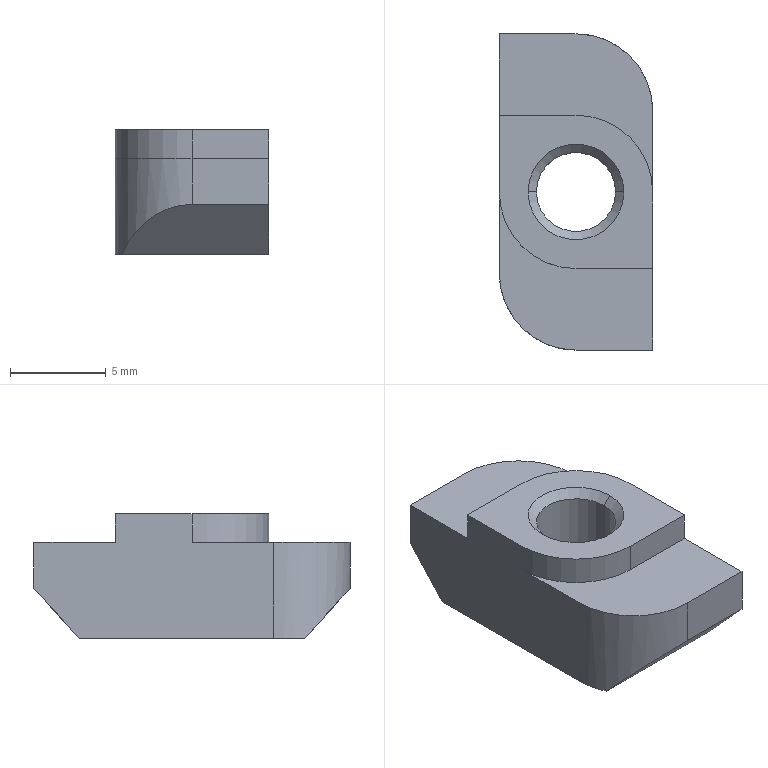Component | SolidWorks | 170423A4-AHC21-308-M5-1 | 1 solid | 22 faces | box 8 x 16.5 x 6.5 mm | volume 584 mm3 | plane 12 | cylinder 6 | cone 4 | commonest cylinder face diameters 8 x4 4.134 x2
STEP:
#1=COLOUR_RGB('',0.7922,0.8196,0.9333);
#2=FILL_AREA_STYLE_COLOUR('',#1);
#3=FILL_AREA_STYLE('',(#2));
#4=SURFACE_STYLE_FILL_AREA(#3);
#5=SURFACE_SIDE_STYLE('',(#4));
#6=SURFACE_STYLE_USAGE(.BOTH.,#5);
#7=PRESENTATION_STYLE_ASSIGNMENT((#6));
#8=CARTESIAN_POINT('',(-7.605,-0.8381,17.989));
#9=VERTEX_POINT('',#8);
#10=CARTESIAN_POINT('',(-7.768,-0.8381,17.989));
#11=VERTEX_POINT('',#10);
#12=CARTESIAN_POINT('',(-7.687,-0.8381,17.989));
#13=DIRECTION('',(0.,0.,-1.));
#14=DIRECTION('',(-1.,0.,0.));
#15=AXIS2_PLACEMENT_3D('',#12,#13,#14);
#16=CIRCLE('',#15,0.08138);
#17=EDGE_CURVE('',#9,#11,#16,.T.);
#18=ORIENTED_EDGE('',*,*,#17,.F.);
#19=CARTESIAN_POINT('',(-7.588,-0.8381,17.972));
#20=VERTEX_POINT('',#19);
#21=CARTESIAN_POINT('',(-7.588,-0.8381,17.972));
#22=DIRECTION('',(0.7071,0.,-0.7071));
#23=VECTOR('',#22,39.37);
#24=LINE('',#21,#23);
#25=EDGE_CURVE('',#9,#20,#24,.T.);
#26=ORIENTED_EDGE('',*,*,#25,.T.);
#27=CARTESIAN_POINT('',(-7.785,-0.8381,17.972));
#28=VERTEX_POINT('',#27);
#29=CARTESIAN_POINT('',(-7.687,-0.8381,17.972));
#30=DIRECTION('',(0.,0.,-1.));
#31=DIRECTION('',(-1.,0.,0.));
#32=AXIS2_PLACEMENT_3D('',#29,#30,#31);
#33=CIRCLE('',#32,0.09843);
#34=EDGE_CURVE('',#20,#28,#33,.T.);
#35=ORIENTED_EDGE('',*,*,#34,.T.);
#36=CARTESIAN_POINT('',(-7.785,-0.8381,17.972));
#37=DIRECTION('',(-0.7071,-0.,-0.7071));
#38=VECTOR('',#37,39.37);
#39=LINE('',#36,#38);
#40=EDGE_CURVE('',#11,#28,#39,.T.);
#41=ORIENTED_EDGE('',*,*,#40,.F.);
#42=EDGE_LOOP('',(#18,#26,#35,#41));
#43=FACE_OUTER_BOUND('',#42,.T.);
#44=CARTESIAN_POINT('',(-7.687,-0.8381,17.972));
#45=DIRECTION('',(0.,0.,-1.));
#46=DIRECTION('',(-1.,0.,0.));
#47=AXIS2_PLACEMENT_3D('',#44,#45,#46);
#48=CONICAL_SURFACE('',#47,0.09843,0.7854);
#49=ADVANCED_FACE('',(#43),#48,.F.);
#50=ORIENTED_EDGE('',*,*,#17,.T.);
#51=CARTESIAN_POINT('',(-7.768,-0.8381,18.211));
#52=VERTEX_POINT('',#51);
#53=CARTESIAN_POINT('',(-7.768,-0.8381,17.972));
#54=DIRECTION('',(-0.,-0.,1.));
#55=VECTOR('',#54,39.37);
#56=LINE('',#53,#55);
#57=EDGE_CURVE('',#11,#52,#56,.T.);
#58=ORIENTED_EDGE('',*,*,#57,.T.);
#59=CARTESIAN_POINT('',(-7.605,-0.8381,18.211));
#60=VERTEX_POINT('',#59);
#61=CARTESIAN_POINT('',(-7.687,-0.8381,18.211));
#62=DIRECTION('',(0.,0.,-1.));
#63=DIRECTION('',(1.,0.,0.));
#64=AXIS2_PLACEMENT_3D('',#61,#62,#63);
#65=CIRCLE('',#64,0.08138);
#66=EDGE_CURVE('',#60,#52,#65,.T.);
#67=ORIENTED_EDGE('',*,*,#66,.F.);
#68=CARTESIAN_POINT('',(-7.605,-0.8381,17.972));
#69=DIRECTION('',(-0.,-0.,1.));
#70=VECTOR('',#69,39.37);
#71=LINE('',#68,#70);
#72=EDGE_CURVE('',#9,#60,#71,.T.);
#73=ORIENTED_EDGE('',*,*,#72,.F.);
#74=EDGE_LOOP('',(#50,#58,#67,#73));
#75=FACE_OUTER_BOUND('',#74,.T.);
#76=CARTESIAN_POINT('',(-7.687,-0.8381,17.972));
#77=DIRECTION('',(-0.,-0.,1.));
#78=DIRECTION('',(1.,0.,0.));
#79=AXIS2_PLACEMENT_3D('',#76,#77,#78);
#80=CYLINDRICAL_SURFACE('',#79,0.08138);
#81=ADVANCED_FACE('',(#75),#80,.F.);
#82=ORIENTED_EDGE('',*,*,#66,.T.);
#83=CARTESIAN_POINT('',(-7.785,-0.8381,18.228));
#84=VERTEX_POINT('',#83);
#85=CARTESIAN_POINT('',(-7.785,-0.8381,18.228));
#86=DIRECTION('',(-0.7071,0.,0.7071));
#87=VECTOR('',#86,39.37);
#88=LINE('',#85,#87);
#89=EDGE_CURVE('',#52,#84,#88,.T.);
#90=ORIENTED_EDGE('',*,*,#89,.T.);
#91=CARTESIAN_POINT('',(-7.588,-0.8381,18.228));
#92=VERTEX_POINT('',#91);
#93=CARTESIAN_POINT('',(-7.687,-0.8381,18.228));
#94=DIRECTION('',(0.,0.,-1.));
#95=DIRECTION('',(1.,0.,0.));
#96=AXIS2_PLACEMENT_3D('',#93,#94,#95);
#97=CIRCLE('',#96,0.09843);
#98=EDGE_CURVE('',#92,#84,#97,.T.);
#99=ORIENTED_EDGE('',*,*,#98,.F.);
#100=CARTESIAN_POINT('',(-7.588,-0.8381,18.228));
#101=DIRECTION('',(0.7071,0.,0.7071));
#102=VECTOR('',#101,39.37);
#103=LINE('',#100,#102);
#104=EDGE_CURVE('',#60,#92,#103,.T.);
#105=ORIENTED_EDGE('',*,*,#104,.F.);
#106=EDGE_LOOP('',(#82,#90,#99,#105));
#107=FACE_OUTER_BOUND('',#106,.T.);
#108=CARTESIAN_POINT('',(-7.687,-0.8381,18.228));
#109=DIRECTION('',(-0.,-0.,1.));
#110=DIRECTION('',(1.,0.,0.));
#111=AXIS2_PLACEMENT_3D('',#108,#109,#110);
#112=CONICAL_SURFACE('',#111,0.09843,0.7854);
#113=ADVANCED_FACE('',(#107),#112,.F.);
#114=CARTESIAN_POINT('',(-7.529,-1.07,17.972));
#115=VERTEX_POINT('',#114);
#116=CARTESIAN_POINT('',(-7.529,-1.163,18.075));
#117=VERTEX_POINT('',#116);
#118=CARTESIAN_POINT('',(-7.529,-1.034,17.933));
#119=DIRECTION('',(0.,-0.6734,0.7393));
#120=VECTOR('',#119,39.37);
#121=LINE('',#118,#120);
#122=EDGE_CURVE('',#115,#117,#121,.T.);
#123=ORIENTED_EDGE('',*,*,#122,.F.);
#124=CARTESIAN_POINT('',(-7.529,-0.6708,17.972));
#125=VERTEX_POINT('',#124);
#126=CARTESIAN_POINT('',(-7.529,-0.6708,17.972));
#127=DIRECTION('',(-0.,1.,0.));
#128=VECTOR('',#127,39.37);
#129=LINE('',#126,#128);
#130=EDGE_CURVE('',#115,#125,#129,.T.);
#131=ORIENTED_EDGE('',*,*,#130,.T.);
#132=CARTESIAN_POINT('',(-7.529,-0.6708,18.169));
#133=VERTEX_POINT('',#132);
#134=CARTESIAN_POINT('',(-7.529,-0.6708,18.169));
#135=DIRECTION('',(0.,0.,-1.));
#136=VECTOR('',#135,39.37);
#137=LINE('',#134,#136);
#138=EDGE_CURVE('',#133,#125,#137,.T.);
#139=ORIENTED_EDGE('',*,*,#138,.F.);
#140=CARTESIAN_POINT('',(-7.529,-0.8381,18.169));
#141=VERTEX_POINT('',#140);
#142=CARTESIAN_POINT('',(-7.529,-1.163,18.169));
#143=DIRECTION('',(-0.,1.,0.));
#144=VECTOR('',#143,39.37);
#145=LINE('',#142,#144);
#146=EDGE_CURVE('',#141,#133,#145,.T.);
#147=ORIENTED_EDGE('',*,*,#146,.F.);
#148=CARTESIAN_POINT('',(-7.529,-0.8381,18.228));
#149=VERTEX_POINT('',#148);
#150=CARTESIAN_POINT('',(-7.529,-0.8381,18.228));
#151=DIRECTION('',(0.,0.,-1.));
#152=VECTOR('',#151,39.37);
#153=LINE('',#150,#152);
#154=EDGE_CURVE('',#149,#141,#153,.T.);
#155=ORIENTED_EDGE('',*,*,#154,.F.);
#156=CARTESIAN_POINT('',(-7.529,-0.9956,18.228));
#157=VERTEX_POINT('',#156);
#158=CARTESIAN_POINT('',(-7.529,-1.163,18.228));
#159=DIRECTION('',(-0.,1.,0.));
#160=VECTOR('',#159,39.37);
#161=LINE('',#158,#160);
#162=EDGE_CURVE('',#157,#149,#161,.T.);
#163=ORIENTED_EDGE('',*,*,#162,.F.);
#164=CARTESIAN_POINT('',(-7.529,-0.9956,18.169));
#165=VERTEX_POINT('',#164);
#166=CARTESIAN_POINT('',(-7.529,-0.9956,18.228));
#167=DIRECTION('',(0.,0.,-1.));
#168=VECTOR('',#167,39.37);
#169=LINE('',#166,#168);
#170=EDGE_CURVE('',#157,#165,#169,.T.);
#171=ORIENTED_EDGE('',*,*,#170,.T.);
#172=CARTESIAN_POINT('',(-7.529,-1.163,18.169));
#173=VERTEX_POINT('',#172);
#174=CARTESIAN_POINT('',(-7.529,-1.163,18.169));
#175=DIRECTION('',(-0.,1.,0.));
#176=VECTOR('',#175,39.37);
#177=LINE('',#174,#176);
#178=EDGE_CURVE('',#173,#165,#177,.T.);
#179=ORIENTED_EDGE('',*,*,#178,.F.);
#180=CARTESIAN_POINT('',(-7.529,-1.163,18.169));
#181=DIRECTION('',(-0.,-0.,1.));
#182=VECTOR('',#181,39.37);
#183=LINE('',#180,#182);
#184=EDGE_CURVE('',#117,#173,#183,.T.);
#185=ORIENTED_EDGE('',*,*,#184,.F.);
#186=EDGE_LOOP('',(#123,#131,#139,#147,#155,#163,#171,#179,#185));
#187=FACE_OUTER_BOUND('',#186,.T.);
#188=CARTESIAN_POINT('',(-7.529,-1.163,18.169));
#189=DIRECTION('',(-1.,-0.,-0.));
#190=DIRECTION('',(0.,-1.,-0.));
#191=AXIS2_PLACEMENT_3D('',#188,#189,#190);
#192=PLANE('',#191);
#193=ADVANCED_FACE('',(#187),#192,.F.);
#194=CARTESIAN_POINT('',(-7.687,-0.8381,17.972));
#195=DIRECTION('',(0.,0.,-1.));
#196=DIRECTION('',(-1.,0.,0.));
#197=AXIS2_PLACEMENT_3D('',#194,#195,#196);
#198=CIRCLE('',#197,0.09843);
#199=EDGE_CURVE('',#28,#20,#198,.T.);
#200=ORIENTED_EDGE('',*,*,#199,.F.);
#201=ORIENTED_EDGE('',*,*,#34,.F.);
#202=EDGE_LOOP('',(#200,#201));
#203=FACE_BOUND('',#202,.T.);
#204=CARTESIAN_POINT('',(-7.844,-0.6066,17.972));
#205=VERTEX_POINT('',#204);
#206=CARTESIAN_POINT('',(-7.844,-1.005,17.972));
#207=VERTEX_POINT('',#206);
#208=CARTESIAN_POINT('',(-7.844,-0.6708,17.972));
#209=DIRECTION('',(0.,-1.,-0.));
#210=VECTOR('',#209,39.37);
#211=LINE('',#208,#210);
#212=EDGE_CURVE('',#205,#207,#211,.T.);
#213=ORIENTED_EDGE('',*,*,#212,.F.);
#214=CARTESIAN_POINT('',(-7.543,-0.6066,17.972));
#215=VERTEX_POINT('',#214);
#216=CARTESIAN_POINT('',(-7.687,-0.6066,17.972));
#217=DIRECTION('',(1.,0.,0.));
#218=VECTOR('',#217,39.37);
#219=LINE('',#216,#218);
#220=EDGE_CURVE('',#205,#215,#219,.T.);
#221=ORIENTED_EDGE('',*,*,#220,.T.);
#222=CARTESIAN_POINT('',(-7.687,-0.6708,17.972));
#223=DIRECTION('',(-0.,-0.,1.));
#224=DIRECTION('',(1.,0.,0.));
#225=AXIS2_PLACEMENT_3D('',#222,#223,#224);
#226=CIRCLE('',#225,0.1575);
#227=EDGE_CURVE('',#125,#215,#226,.T.);
#228=ORIENTED_EDGE('',*,*,#227,.F.);
#229=ORIENTED_EDGE('',*,*,#130,.F.);
#230=CARTESIAN_POINT('',(-7.831,-1.07,17.972));
#231=VERTEX_POINT('',#230);
#232=CARTESIAN_POINT('',(-7.687,-1.07,17.972));
#233=DIRECTION('',(-1.,-0.,-0.));
#234=VECTOR('',#233,39.37);
#235=LINE('',#232,#234);
#236=EDGE_CURVE('',#115,#231,#235,.T.);
#237=ORIENTED_EDGE('',*,*,#236,.T.);
#238=CARTESIAN_POINT('',(-7.687,-1.005,17.972));
#239=DIRECTION('',(-0.,-0.,1.));
#240=DIRECTION('',(1.,0.,0.));
#241=AXIS2_PLACEMENT_3D('',#238,#239,#240);
#242=CIRCLE('',#241,0.1575);
#243=EDGE_CURVE('',#207,#231,#242,.T.);
#244=ORIENTED_EDGE('',*,*,#243,.F.);
#245=EDGE_LOOP('',(#213,#221,#228,#229,#237,#244));
#246=FACE_OUTER_BOUND('',#245,.T.);
#247=CARTESIAN_POINT('',(-7.687,-0.6708,17.972));
#248=DIRECTION('',(-0.,-0.,1.));
#249=DIRECTION('',(1.,0.,0.));
#250=AXIS2_PLACEMENT_3D('',#247,#248,#249);
#251=PLANE('',#250);
#252=ADVANCED_FACE('',(#203,#246),#251,.F.);
#253=ORIENTED_EDGE('',*,*,#25,.F.);
#254=CARTESIAN_POINT('',(-7.687,-0.8381,17.989));
#255=DIRECTION('',(0.,0.,-1.));
#256=DIRECTION('',(-1.,0.,0.));
#257=AXIS2_PLACEMENT_3D('',#254,#255,#256);
#258=CIRCLE('',#257,0.08138);
#259=EDGE_CURVE('',#11,#9,#258,.T.);
#260=ORIENTED_EDGE('',*,*,#259,.F.);
#261=ORIENTED_EDGE('',*,*,#40,.T.);
#262=ORIENTED_EDGE('',*,*,#199,.T.);
#263=EDGE_LOOP('',(#253,#260,#261,#262));
#264=FACE_OUTER_BOUND('',#263,.T.);
#265=CARTESIAN_POINT('',(-7.687,-0.8381,17.972));
#266=DIRECTION('',(0.,0.,-1.));
#267=DIRECTION('',(-1.,0.,0.));
#268=AXIS2_PLACEMENT_3D('',#265,#266,#267);
#269=CONICAL_SURFACE('',#268,0.09843,0.7854);
#270=ADVANCED_FACE('',(#264),#269,.F.);
#271=CARTESIAN_POINT('',(-7.844,-0.5133,18.075));
#272=VERTEX_POINT('',#271);
#273=CARTESIAN_POINT('',(-7.844,-0.5133,18.169));
#274=VERTEX_POINT('',#273);
#275=CARTESIAN_POINT('',(-7.844,-0.5133,18.169));
#276=DIRECTION('',(-0.,-0.,1.));
#277=VECTOR('',#276,39.37);
#278=LINE('',#275,#277);
#279=EDGE_CURVE('',#272,#274,#278,.T.);
#280=ORIENTED_EDGE('',*,*,#279,.F.);
#281=CARTESIAN_POINT('',(-7.844,-0.4775,18.114));
#282=DIRECTION('',(0.,-0.6734,-0.7393));
#283=VECTOR('',#282,39.37);
#284=LINE('',#281,#283);
#285=EDGE_CURVE('',#272,#205,#284,.T.);
#286=ORIENTED_EDGE('',*,*,#285,.T.);
#287=ORIENTED_EDGE('',*,*,#212,.T.);
#288=CARTESIAN_POINT('',(-7.844,-1.005,18.169));
#289=VERTEX_POINT('',#288);
#290=CARTESIAN_POINT('',(-7.844,-1.005,18.169));
#291=DIRECTION('',(0.,0.,-1.));
#292=VECTOR('',#291,39.37);
#293=LINE('',#290,#292);
#294=EDGE_CURVE('',#289,#207,#293,.T.);
#295=ORIENTED_EDGE('',*,*,#294,.F.);
#296=CARTESIAN_POINT('',(-7.844,-0.8381,18.169));
#297=VERTEX_POINT('',#296);
#298=CARTESIAN_POINT('',(-7.844,-0.5133,18.169));
#299=DIRECTION('',(-0.,-1.,-0.));
#300=VECTOR('',#299,39.37);
#301=LINE('',#298,#300);
#302=EDGE_CURVE('',#297,#289,#301,.T.);
#303=ORIENTED_EDGE('',*,*,#302,.F.);
#304=CARTESIAN_POINT('',(-7.844,-0.8381,18.228));
#305=VERTEX_POINT('',#304);
#306=CARTESIAN_POINT('',(-7.844,-0.8381,18.228));
#307=DIRECTION('',(0.,0.,-1.));
#308=VECTOR('',#307,39.37);
#309=LINE('',#306,#308);
#310=EDGE_CURVE('',#305,#297,#309,.T.);
#311=ORIENTED_EDGE('',*,*,#310,.F.);
#312=CARTESIAN_POINT('',(-7.844,-0.6806,18.228));
#313=VERTEX_POINT('',#312);
#314=CARTESIAN_POINT('',(-7.844,-0.5133,18.228));
#315=DIRECTION('',(-0.,-1.,-0.));
#316=VECTOR('',#315,39.37);
#317=LINE('',#314,#316);
#318=EDGE_CURVE('',#313,#305,#317,.T.);
#319=ORIENTED_EDGE('',*,*,#318,.F.);
#320=CARTESIAN_POINT('',(-7.844,-0.6806,18.169));
#321=VERTEX_POINT('',#320);
#322=CARTESIAN_POINT('',(-7.844,-0.6806,18.228));
#323=DIRECTION('',(0.,0.,-1.));
#324=VECTOR('',#323,39.37);
#325=LINE('',#322,#324);
#326=EDGE_CURVE('',#313,#321,#325,.T.);
#327=ORIENTED_EDGE('',*,*,#326,.T.);
#328=CARTESIAN_POINT('',(-7.844,-0.5133,18.169));
#329=DIRECTION('',(-0.,-1.,-0.));
#330=VECTOR('',#329,39.37);
#331=LINE('',#328,#330);
#332=EDGE_CURVE('',#274,#321,#331,.T.);
#333=ORIENTED_EDGE('',*,*,#332,.F.);
#334=EDGE_LOOP('',(#280,#286,#287,#295,#303,#311,#319,#327,#333));
#335=FACE_OUTER_BOUND('',#334,.T.);
#336=CARTESIAN_POINT('',(-7.844,-0.5133,18.169));
#337=DIRECTION('',(1.,-0.,0.));
#338=DIRECTION('',(0.,1.,0.));
#339=AXIS2_PLACEMENT_3D('',#336,#337,#338);
#340=PLANE('',#339);
#341=ADVANCED_FACE('',(#335),#340,.F.);
#342=CARTESIAN_POINT('',(-7.687,-0.5133,18.075));
#343=VERTEX_POINT('',#342);
#344=CARTESIAN_POINT('',(-7.687,-0.5133,18.075));
#345=CARTESIAN_POINT('',(-7.623,-0.5133,18.075));
#346=CARTESIAN_POINT('',(-7.569,-0.5481,18.037));
#347=CARTESIAN_POINT('',(-7.543,-0.6066,17.972));
#348=(BOUNDED_CURVE()B_SPLINE_CURVE(3,(#344,#345,#346,#347),.UNSPECIFIED.,.F.,.T.)B_SPLINE_CURVE_WITH_KNOTS((4,4),(0.,1.151),.UNSPECIFIED.)CURVE()GEOMETRIC_REPRESENTATION_ITEM()RATIONAL_B_SPLINE_CURVE((1.,0.8927,0.8927,1.))REPRESENTATION_ITEM(''));
#349=EDGE_CURVE('',#343,#215,#348,.T.);
#350=ORIENTED_EDGE('',*,*,#349,.F.);
#351=CARTESIAN_POINT('',(-7.687,-0.5133,18.169));
#352=VERTEX_POINT('',#351);
#353=CARTESIAN_POINT('',(-7.687,-0.5133,18.169));
#354=DIRECTION('',(-0.,-0.,1.));
#355=VECTOR('',#354,39.37);
#356=LINE('',#353,#355);
#357=EDGE_CURVE('',#343,#352,#356,.T.);
#358=ORIENTED_EDGE('',*,*,#357,.T.);
#359=CARTESIAN_POINT('',(-7.687,-0.6708,18.169));
#360=DIRECTION('',(0.,0.,-1.));
#361=DIRECTION('',(1.,0.,0.));
#362=AXIS2_PLACEMENT_3D('',#359,#360,#361);
#363=CIRCLE('',#362,0.1575);
#364=EDGE_CURVE('',#352,#133,#363,.T.);
#365=ORIENTED_EDGE('',*,*,#364,.T.);
#366=ORIENTED_EDGE('',*,*,#138,.T.);
#367=ORIENTED_EDGE('',*,*,#227,.T.);
#368=EDGE_LOOP('',(#350,#358,#365,#366,#367));
#369=FACE_OUTER_BOUND('',#368,.T.);
#370=CARTESIAN_POINT('',(-7.687,-0.6708,18.169));
#371=DIRECTION('',(-0.,-0.,1.));
#372=DIRECTION('',(1.,0.,0.));
#373=AXIS2_PLACEMENT_3D('',#370,#371,#372);
#374=CYLINDRICAL_SURFACE('',#373,0.1575);
#375=ADVANCED_FACE('',(#369),#374,.T.);
#376=CARTESIAN_POINT('',(-7.687,-1.163,18.075));
#377=VERTEX_POINT('',#376);
#378=CARTESIAN_POINT('',(-7.687,-1.163,18.075));
#379=CARTESIAN_POINT('',(-7.751,-1.163,18.075));
#380=CARTESIAN_POINT('',(-7.805,-1.128,18.037));
#381=CARTESIAN_POINT('',(-7.831,-1.07,17.972));
#382=(BOUNDED_CURVE()B_SPLINE_CURVE(3,(#378,#379,#380,#381),.UNSPECIFIED.,.F.,.T.)B_SPLINE_CURVE_WITH_KNOTS((4,4),(0.,1.151),.UNSPECIFIED.)CURVE()GEOMETRIC_REPRESENTATION_ITEM()RATIONAL_B_SPLINE_CURVE((1.,0.8927,0.8927,1.))REPRESENTATION_ITEM(''));
#383=EDGE_CURVE('',#377,#231,#382,.T.);
#384=ORIENTED_EDGE('',*,*,#383,.F.);
#385=CARTESIAN_POINT('',(-7.687,-1.163,18.169));
#386=VERTEX_POINT('',#385);
#387=CARTESIAN_POINT('',(-7.687,-1.163,18.169));
#388=DIRECTION('',(-0.,-0.,1.));
#389=VECTOR('',#388,39.37);
#390=LINE('',#387,#389);
#391=EDGE_CURVE('',#377,#386,#390,.T.);
#392=ORIENTED_EDGE('',*,*,#391,.T.);
#393=CARTESIAN_POINT('',(-7.687,-1.005,18.169));
#394=DIRECTION('',(0.,0.,-1.));
#395=DIRECTION('',(1.,0.,0.));
#396=AXIS2_PLACEMENT_3D('',#393,#394,#395);
#397=CIRCLE('',#396,0.1575);
#398=EDGE_CURVE('',#386,#289,#397,.T.);
#399=ORIENTED_EDGE('',*,*,#398,.T.);
#400=ORIENTED_EDGE('',*,*,#294,.T.);
#401=ORIENTED_EDGE('',*,*,#243,.T.);
#402=EDGE_LOOP('',(#384,#392,#399,#400,#401));
#403=FACE_OUTER_BOUND('',#402,.T.);
#404=CARTESIAN_POINT('',(-7.687,-1.005,18.169));
#405=DIRECTION('',(-0.,-0.,1.));
#406=DIRECTION('',(1.,0.,0.));
#407=AXIS2_PLACEMENT_3D('',#404,#405,#406);
#408=CYLINDRICAL_SURFACE('',#407,0.1575);
#409=ADVANCED_FACE('',(#403),#408,.T.);
#410=ORIENTED_EDGE('',*,*,#57,.F.);
#411=ORIENTED_EDGE('',*,*,#259,.T.);
#412=ORIENTED_EDGE('',*,*,#72,.T.);
#413=CARTESIAN_POINT('',(-7.687,-0.8381,18.211));
#414=DIRECTION('',(0.,0.,-1.));
#415=DIRECTION('',(1.,0.,0.));
#416=AXIS2_PLACEMENT_3D('',#413,#414,#415);
#417=CIRCLE('',#416,0.08138);
#418=EDGE_CURVE('',#52,#60,#417,.T.);
#419=ORIENTED_EDGE('',*,*,#418,.F.);
#420=EDGE_LOOP('',(#410,#411,#412,#419));
#421=FACE_OUTER_BOUND('',#420,.T.);
#422=CARTESIAN_POINT('',(-7.687,-0.8381,17.972));
#423=DIRECTION('',(-0.,-0.,1.));
#424=DIRECTION('',(1.,0.,0.));
#425=AXIS2_PLACEMENT_3D('',#422,#423,#424);
#426=CYLINDRICAL_SURFACE('',#425,0.08138);
#427=ADVANCED_FACE('',(#421),#426,.F.);
#428=ORIENTED_EDGE('',*,*,#357,.F.);
#429=CARTESIAN_POINT('',(-7.687,-0.5133,18.075));
#430=DIRECTION('',(-1.,-0.,-0.));
#431=VECTOR('',#430,39.37);
#432=LINE('',#429,#431);
#433=EDGE_CURVE('',#343,#272,#432,.T.);
#434=ORIENTED_EDGE('',*,*,#433,.T.);
#435=ORIENTED_EDGE('',*,*,#279,.T.);
#436=CARTESIAN_POINT('',(-7.687,-0.5133,18.169));
#437=DIRECTION('',(-1.,-0.,-0.));
#438=VECTOR('',#437,39.37);
#439=LINE('',#436,#438);
#440=EDGE_CURVE('',#352,#274,#439,.T.);
#441=ORIENTED_EDGE('',*,*,#440,.F.);
#442=EDGE_LOOP('',(#428,#434,#435,#441));
#443=FACE_OUTER_BOUND('',#442,.T.);
#444=CARTESIAN_POINT('',(-7.687,-0.5133,18.169));
#445=DIRECTION('',(0.,-1.,-0.));
#446=DIRECTION('',(1.,0.,0.));
#447=AXIS2_PLACEMENT_3D('',#444,#445,#446);
#448=PLANE('',#447);
#449=ADVANCED_FACE('',(#443),#448,.F.);
#450=CARTESIAN_POINT('',(-7.687,-1.163,18.169));
#451=DIRECTION('',(1.,0.,0.));
#452=VECTOR('',#451,39.37);
#453=LINE('',#450,#452);
#454=EDGE_CURVE('',#386,#173,#453,.T.);
#455=ORIENTED_EDGE('',*,*,#454,.T.);
#456=ORIENTED_EDGE('',*,*,#178,.T.);
#457=CARTESIAN_POINT('',(-7.687,-0.9956,18.169));
#458=VERTEX_POINT('',#457);
#459=CARTESIAN_POINT('',(-7.687,-0.9956,18.169));
#460=DIRECTION('',(-1.,-0.,-0.));
#461=VECTOR('',#460,39.37);
#462=LINE('',#459,#461);
#463=EDGE_CURVE('',#165,#458,#462,.T.);
#464=ORIENTED_EDGE('',*,*,#463,.T.);
#465=CARTESIAN_POINT('',(-7.687,-0.8381,18.169));
#466=DIRECTION('',(0.,0.,-1.));
#467=DIRECTION('',(1.,0.,0.));
#468=AXIS2_PLACEMENT_3D('',#465,#466,#467);
#469=CIRCLE('',#468,0.1575);
#470=EDGE_CURVE('',#458,#297,#469,.T.);
#471=ORIENTED_EDGE('',*,*,#470,.T.);
#472=ORIENTED_EDGE('',*,*,#302,.T.);
#473=ORIENTED_EDGE('',*,*,#398,.F.);
#474=EDGE_LOOP('',(#455,#456,#464,#471,#472,#473));
#475=FACE_OUTER_BOUND('',#474,.T.);
#476=CARTESIAN_POINT('',(-7.687,-0.6708,18.169));
#477=DIRECTION('',(-0.,-0.,1.));
#478=DIRECTION('',(1.,0.,0.));
#479=AXIS2_PLACEMENT_3D('',#476,#477,#478);
#480=PLANE('',#479);
#481=ADVANCED_FACE('',(#475),#480,.T.);
#482=ORIENTED_EDGE('',*,*,#98,.T.);
#483=CARTESIAN_POINT('',(-7.687,-0.8381,18.228));
#484=DIRECTION('',(0.,0.,-1.));
#485=DIRECTION('',(1.,0.,0.));
#486=AXIS2_PLACEMENT_3D('',#483,#484,#485);
#487=CIRCLE('',#486,0.09843);
#488=EDGE_CURVE('',#84,#92,#487,.T.);
#489=ORIENTED_EDGE('',*,*,#488,.T.);
#490=EDGE_LOOP('',(#482,#489));
#491=FACE_BOUND('',#490,.T.);
#492=ORIENTED_EDGE('',*,*,#318,.T.);
#493=CARTESIAN_POINT('',(-7.687,-0.9956,18.228));
#494=VERTEX_POINT('',#493);
#495=CARTESIAN_POINT('',(-7.687,-0.8381,18.228));
#496=DIRECTION('',(-0.,-0.,1.));
#497=DIRECTION('',(1.,0.,0.));
#498=AXIS2_PLACEMENT_3D('',#495,#496,#497);
#499=CIRCLE('',#498,0.1575);
#500=EDGE_CURVE('',#305,#494,#499,.T.);
#501=ORIENTED_EDGE('',*,*,#500,.T.);
#502=CARTESIAN_POINT('',(-7.687,-0.9956,18.228));
#503=DIRECTION('',(1.,0.,0.));
#504=VECTOR('',#503,39.37);
#505=LINE('',#502,#504);
#506=EDGE_CURVE('',#494,#157,#505,.T.);
#507=ORIENTED_EDGE('',*,*,#506,.T.);
#508=ORIENTED_EDGE('',*,*,#162,.T.);
#509=CARTESIAN_POINT('',(-7.687,-0.6806,18.228));
#510=VERTEX_POINT('',#509);
#511=CARTESIAN_POINT('',(-7.687,-0.8381,18.228));
#512=DIRECTION('',(-0.,-0.,1.));
#513=DIRECTION('',(1.,0.,0.));
#514=AXIS2_PLACEMENT_3D('',#511,#512,#513);
#515=CIRCLE('',#514,0.1575);
#516=EDGE_CURVE('',#149,#510,#515,.T.);
#517=ORIENTED_EDGE('',*,*,#516,.T.);
#518=CARTESIAN_POINT('',(-7.687,-0.6806,18.228));
#519=DIRECTION('',(-1.,-0.,-0.));
#520=VECTOR('',#519,39.37);
#521=LINE('',#518,#520);
#522=EDGE_CURVE('',#510,#313,#521,.T.);
#523=ORIENTED_EDGE('',*,*,#522,.T.);
#524=EDGE_LOOP('',(#492,#501,#507,#508,#517,#523));
#525=FACE_OUTER_BOUND('',#524,.T.);
#526=CARTESIAN_POINT('',(-7.687,-0.8381,18.228));
#527=DIRECTION('',(-0.,-0.,1.));
#528=DIRECTION('',(1.,0.,0.));
#529=AXIS2_PLACEMENT_3D('',#526,#527,#528);
#530=PLANE('',#529);
#531=ADVANCED_FACE('',(#491,#525),#530,.T.);
#532=ORIENTED_EDGE('',*,*,#440,.T.);
#533=ORIENTED_EDGE('',*,*,#332,.T.);
#534=CARTESIAN_POINT('',(-7.687,-0.6806,18.169));
#535=VERTEX_POINT('',#534);
#536=CARTESIAN_POINT('',(-7.687,-0.6806,18.169));
#537=DIRECTION('',(1.,0.,0.));
#538=VECTOR('',#537,39.37);
#539=LINE('',#536,#538);
#540=EDGE_CURVE('',#321,#535,#539,.T.);
#541=ORIENTED_EDGE('',*,*,#540,.T.);
#542=CARTESIAN_POINT('',(-7.687,-0.8381,18.169));
#543=DIRECTION('',(0.,0.,-1.));
#544=DIRECTION('',(1.,0.,0.));
#545=AXIS2_PLACEMENT_3D('',#542,#543,#544);
#546=CIRCLE('',#545,0.1575);
#547=EDGE_CURVE('',#535,#141,#546,.T.);
#548=ORIENTED_EDGE('',*,*,#547,.T.);
#549=ORIENTED_EDGE('',*,*,#146,.T.);
#550=ORIENTED_EDGE('',*,*,#364,.F.);
#551=EDGE_LOOP('',(#532,#533,#541,#548,#549,#550));
#552=FACE_OUTER_BOUND('',#551,.T.);
#553=CARTESIAN_POINT('',(-7.687,-0.6708,18.169));
#554=DIRECTION('',(-0.,-0.,1.));
#555=DIRECTION('',(1.,0.,0.));
#556=AXIS2_PLACEMENT_3D('',#553,#554,#555);
#557=PLANE('',#556);
#558=ADVANCED_FACE('',(#552),#557,.T.);
#559=ORIENTED_EDGE('',*,*,#391,.F.);
#560=CARTESIAN_POINT('',(-7.687,-1.163,18.075));
#561=DIRECTION('',(1.,0.,0.));
#562=VECTOR('',#561,39.37);
#563=LINE('',#560,#562);
#564=EDGE_CURVE('',#377,#117,#563,.T.);
#565=ORIENTED_EDGE('',*,*,#564,.T.);
#566=ORIENTED_EDGE('',*,*,#184,.T.);
#567=ORIENTED_EDGE('',*,*,#454,.F.);
#568=EDGE_LOOP('',(#559,#565,#566,#567));
#569=FACE_OUTER_BOUND('',#568,.T.);
#570=CARTESIAN_POINT('',(-7.687,-1.163,18.169));
#571=DIRECTION('',(-0.,1.,0.));
#572=DIRECTION('',(-1.,-0.,-0.));
#573=AXIS2_PLACEMENT_3D('',#570,#571,#572);
#574=PLANE('',#573);
#575=ADVANCED_FACE('',(#569),#574,.F.);
#576=ORIENTED_EDGE('',*,*,#89,.F.);
#577=ORIENTED_EDGE('',*,*,#418,.T.);
#578=ORIENTED_EDGE('',*,*,#104,.T.);
#579=ORIENTED_EDGE('',*,*,#488,.F.);
#580=EDGE_LOOP('',(#576,#577,#578,#579));
#581=FACE_OUTER_BOUND('',#580,.T.);
#582=CARTESIAN_POINT('',(-7.687,-0.8381,18.228));
#583=DIRECTION('',(-0.,-0.,1.));
#584=DIRECTION('',(1.,0.,0.));
#585=AXIS2_PLACEMENT_3D('',#582,#583,#584);
#586=CONICAL_SURFACE('',#585,0.09843,0.7854);
#587=ADVANCED_FACE('',(#581),#586,.F.);
#588=ORIENTED_EDGE('',*,*,#500,.F.);
#589=ORIENTED_EDGE('',*,*,#310,.T.);
#590=ORIENTED_EDGE('',*,*,#470,.F.);
#591=CARTESIAN_POINT('',(-7.687,-0.9956,18.228));
#592=DIRECTION('',(-0.,-0.,1.));
#593=VECTOR('',#592,39.37);
#594=LINE('',#591,#593);
#595=EDGE_CURVE('',#458,#494,#594,.T.);
#596=ORIENTED_EDGE('',*,*,#595,.T.);
#597=EDGE_LOOP('',(#588,#589,#590,#596));
#598=FACE_OUTER_BOUND('',#597,.T.);
#599=CARTESIAN_POINT('',(-7.687,-0.8381,18.228));
#600=DIRECTION('',(-0.,-0.,1.));
#601=DIRECTION('',(1.,0.,0.));
#602=AXIS2_PLACEMENT_3D('',#599,#600,#601);
#603=CYLINDRICAL_SURFACE('',#602,0.1575);
#604=ADVANCED_FACE('',(#598),#603,.T.);
#605=ORIENTED_EDGE('',*,*,#170,.F.);
#606=ORIENTED_EDGE('',*,*,#506,.F.);
#607=ORIENTED_EDGE('',*,*,#595,.F.);
#608=ORIENTED_EDGE('',*,*,#463,.F.);
#609=EDGE_LOOP('',(#605,#606,#607,#608));
#610=FACE_OUTER_BOUND('',#609,.T.);
#611=CARTESIAN_POINT('',(-7.687,-0.9956,18.228));
#612=DIRECTION('',(-0.,1.,0.));
#613=DIRECTION('',(-1.,-0.,-0.));
#614=AXIS2_PLACEMENT_3D('',#611,#612,#613);
#615=PLANE('',#614);
#616=ADVANCED_FACE('',(#610),#615,.F.);
#617=ORIENTED_EDGE('',*,*,#326,.F.);
#618=ORIENTED_EDGE('',*,*,#522,.F.);
#619=CARTESIAN_POINT('',(-7.687,-0.6806,18.228));
#620=DIRECTION('',(-0.,-0.,1.));
#621=VECTOR('',#620,39.37);
#622=LINE('',#619,#621);
#623=EDGE_CURVE('',#535,#510,#622,.T.);
#624=ORIENTED_EDGE('',*,*,#623,.F.);
#625=ORIENTED_EDGE('',*,*,#540,.F.);
#626=EDGE_LOOP('',(#617,#618,#624,#625));
#627=FACE_OUTER_BOUND('',#626,.T.);
#628=CARTESIAN_POINT('',(-7.687,-0.6806,18.228));
#629=DIRECTION('',(0.,-1.,-0.));
#630=DIRECTION('',(1.,0.,0.));
#631=AXIS2_PLACEMENT_3D('',#628,#629,#630);
#632=PLANE('',#631);
#633=ADVANCED_FACE('',(#627),#632,.F.);
#634=ORIENTED_EDGE('',*,*,#516,.F.);
#635=ORIENTED_EDGE('',*,*,#154,.T.);
#636=ORIENTED_EDGE('',*,*,#547,.F.);
#637=ORIENTED_EDGE('',*,*,#623,.T.);
#638=EDGE_LOOP('',(#634,#635,#636,#637));
#639=FACE_OUTER_BOUND('',#638,.T.);
#640=CARTESIAN_POINT('',(-7.687,-0.8381,18.228));
#641=DIRECTION('',(-0.,-0.,1.));
#642=DIRECTION('',(1.,0.,0.));
#643=AXIS2_PLACEMENT_3D('',#640,#641,#642);
#644=CYLINDRICAL_SURFACE('',#643,0.1575);
#645=ADVANCED_FACE('',(#639),#644,.T.);
#646=ORIENTED_EDGE('',*,*,#383,.T.);
#647=ORIENTED_EDGE('',*,*,#236,.F.);
#648=ORIENTED_EDGE('',*,*,#122,.T.);
#649=ORIENTED_EDGE('',*,*,#564,.F.);
#650=EDGE_LOOP('',(#646,#647,#648,#649));
#651=FACE_OUTER_BOUND('',#650,.T.);
#652=CARTESIAN_POINT('',(-7.844,-1.034,17.933));
#653=DIRECTION('',(-0.,0.7393,0.6734));
#654=DIRECTION('',(0.,-0.6734,0.7393));
#655=AXIS2_PLACEMENT_3D('',#652,#653,#654);
#656=PLANE('',#655);
#657=ADVANCED_FACE('',(#651),#656,.F.);
#658=ORIENTED_EDGE('',*,*,#349,.T.);
#659=ORIENTED_EDGE('',*,*,#220,.F.);
#660=ORIENTED_EDGE('',*,*,#285,.F.);
#661=ORIENTED_EDGE('',*,*,#433,.F.);
#662=EDGE_LOOP('',(#658,#659,#660,#661));
#663=FACE_OUTER_BOUND('',#662,.T.);
#664=CARTESIAN_POINT('',(-7.844,-0.6424,17.933));
#665=DIRECTION('',(0.,-0.7393,0.6734));
#666=DIRECTION('',(0.,-0.6734,-0.7393));
#667=AXIS2_PLACEMENT_3D('',#664,#665,#666);
#668=PLANE('',#667);
#669=ADVANCED_FACE('',(#663),#668,.F.);
#670=CLOSED_SHELL('',(#49,#81,#113,#193,#252,#270,#341,#375,#409,#427,#449,#481,#531,#558,#575,#587,#604,#616,#633,#645,#657,#669));
#671=MANIFOLD_SOLID_BREP('',#670);
#672=STYLED_ITEM('',(#7),#671);
#673=(LENGTH_UNIT()NAMED_UNIT(*)SI_UNIT($,.METRE.));
#674=LENGTH_MEASURE_WITH_UNIT(LENGTH_MEASURE(0.0254),#673);
#675=DIMENSIONAL_EXPONENTS(1.,0.,0.,0.,0.,0.,0.);
#676=(CONVERSION_BASED_UNIT('',#674)LENGTH_UNIT()NAMED_UNIT(#675));
#677=UNCERTAINTY_MEASURE_WITH_UNIT(LENGTH_MEASURE(0.00001),#676,'','');
#678=(NAMED_UNIT(*)PLANE_ANGLE_UNIT()SI_UNIT($,.RADIAN.));
#679=(NAMED_UNIT(*)SI_UNIT($,.STERADIAN.)SOLID_ANGLE_UNIT());
#680=(GEOMETRIC_REPRESENTATION_CONTEXT(3)GLOBAL_UNCERTAINTY_ASSIGNED_CONTEXT((#677))GLOBAL_UNIT_ASSIGNED_CONTEXT((#676,#678,#679))REPRESENTATION_CONTEXT('',''));
#681=MECHANICAL_DESIGN_GEOMETRIC_PRESENTATION_REPRESENTATION('',(#672),#680);
#682=PRESENTATION_LAYER_ASSIGNMENT('','',(#672));
#683=CARTESIAN_POINT('',(0.,0.,0.));
#684=DIRECTION('',(0.,0.,1.));
#685=DIRECTION('',(1.,0.,0.));
#686=AXIS2_PLACEMENT_3D('',#683,#684,#685);
#687=(LENGTH_UNIT()NAMED_UNIT(*)SI_UNIT($,.METRE.));
#688=LENGTH_MEASURE_WITH_UNIT(LENGTH_MEASURE(0.0254),#687);
#689=DIMENSIONAL_EXPONENTS(1.,0.,0.,0.,0.,0.,0.);
#690=(CONVERSION_BASED_UNIT('',#688)LENGTH_UNIT()NAMED_UNIT(#689));
#691=UNCERTAINTY_MEASURE_WITH_UNIT(LENGTH_MEASURE(0.00001),#690,'','');
#692=(NAMED_UNIT(*)PLANE_ANGLE_UNIT()SI_UNIT($,.RADIAN.));
#693=(NAMED_UNIT(*)SI_UNIT($,.STERADIAN.)SOLID_ANGLE_UNIT());
#694=(GEOMETRIC_REPRESENTATION_CONTEXT(3)GLOBAL_UNCERTAINTY_ASSIGNED_CONTEXT((#691))GLOBAL_UNIT_ASSIGNED_CONTEXT((#690,#692,#693))REPRESENTATION_CONTEXT('',''));
#695=ADVANCED_BREP_SHAPE_REPRESENTATION('',(#671,#686),#694);